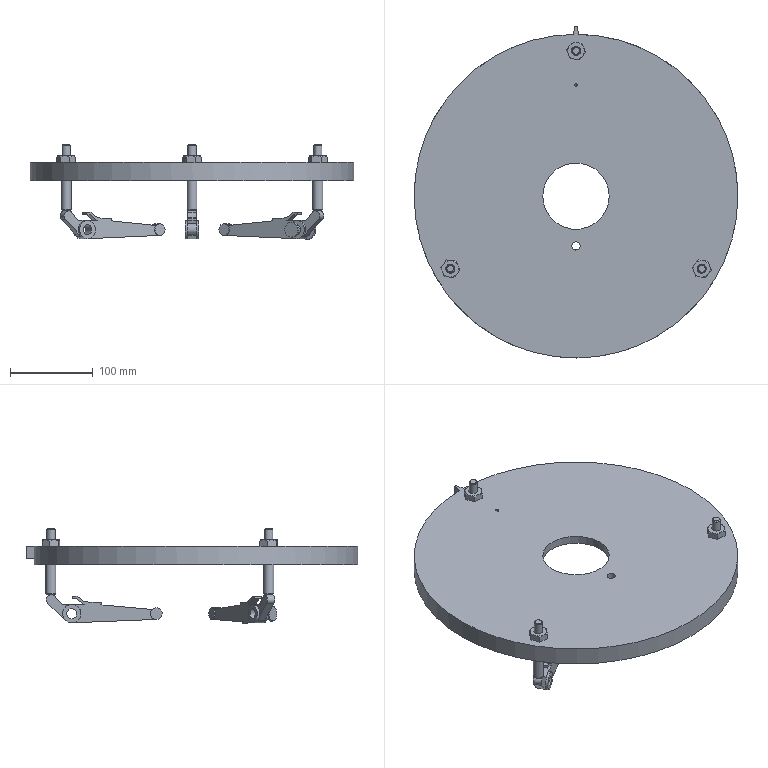Assembly | NX | mm | 12 component files | 12 solids | 175 faces | box 390 x 400.01 x 114.76 mm | volume 2108076 mm3 | plane 110 | cylinder 39 | cone 25 | torus 1 | commonest cylinder face diameters 12 x13 10 x4 14 x3 22 x3 12.5 x3 11 x3 3.2 x2 240 x1
Bill of materials:
unnamed part 1 | 3 |  | Hexagonal prism with a central through-bore; one face has chamfered corners, giving it the shape of a hex nut.
unnamed part 2 | 1 |  | Straight cylindrical pin with a flat disc-shaped head at one end, a chamfered or rounded opposite end, and a smaller cylindrical cross pin passing through the shank near that end.
unnamed part 3 | 1 |  | Thin flat circular plate with a large central hole, several small through-holes, and a small tab sticking out of the outer edge.
unnamed part 4 | 3 |  | Stepped solid cylindrical pin with two coaxial sections of different diameter and chamfered ends.
unnamed part 5 | 3 |  | Lever-like arm: a tapered flat body with a bored cylindrical hub near one end, an angled arm rising from that hub to a rounded cylindrical boss, a cylindrical boss at the opposite tapered end, and a small raised tab or hook on the top edge.
unnamed part 6 | 1 |  | Plain flat annular ring (washer-like) with a central through-hole and square edges.
Mates:
1. fix | Drivingflange 1 component
2. concentric | HexnutM12 3 edge | Drivingflange 1 edge
3. fix | assembly component
4. bond | HexnutM12 3 component | assembly component
5. bond | HexnutM12 2 component | assembly component
6. bond | HexnutM12 1 component | assembly component
7. circular | assembly datumaxis | assembly cartesiancoordinatesystem | assembly cartesiancoordinatesystem | assembly cartesiancoordinatesystem